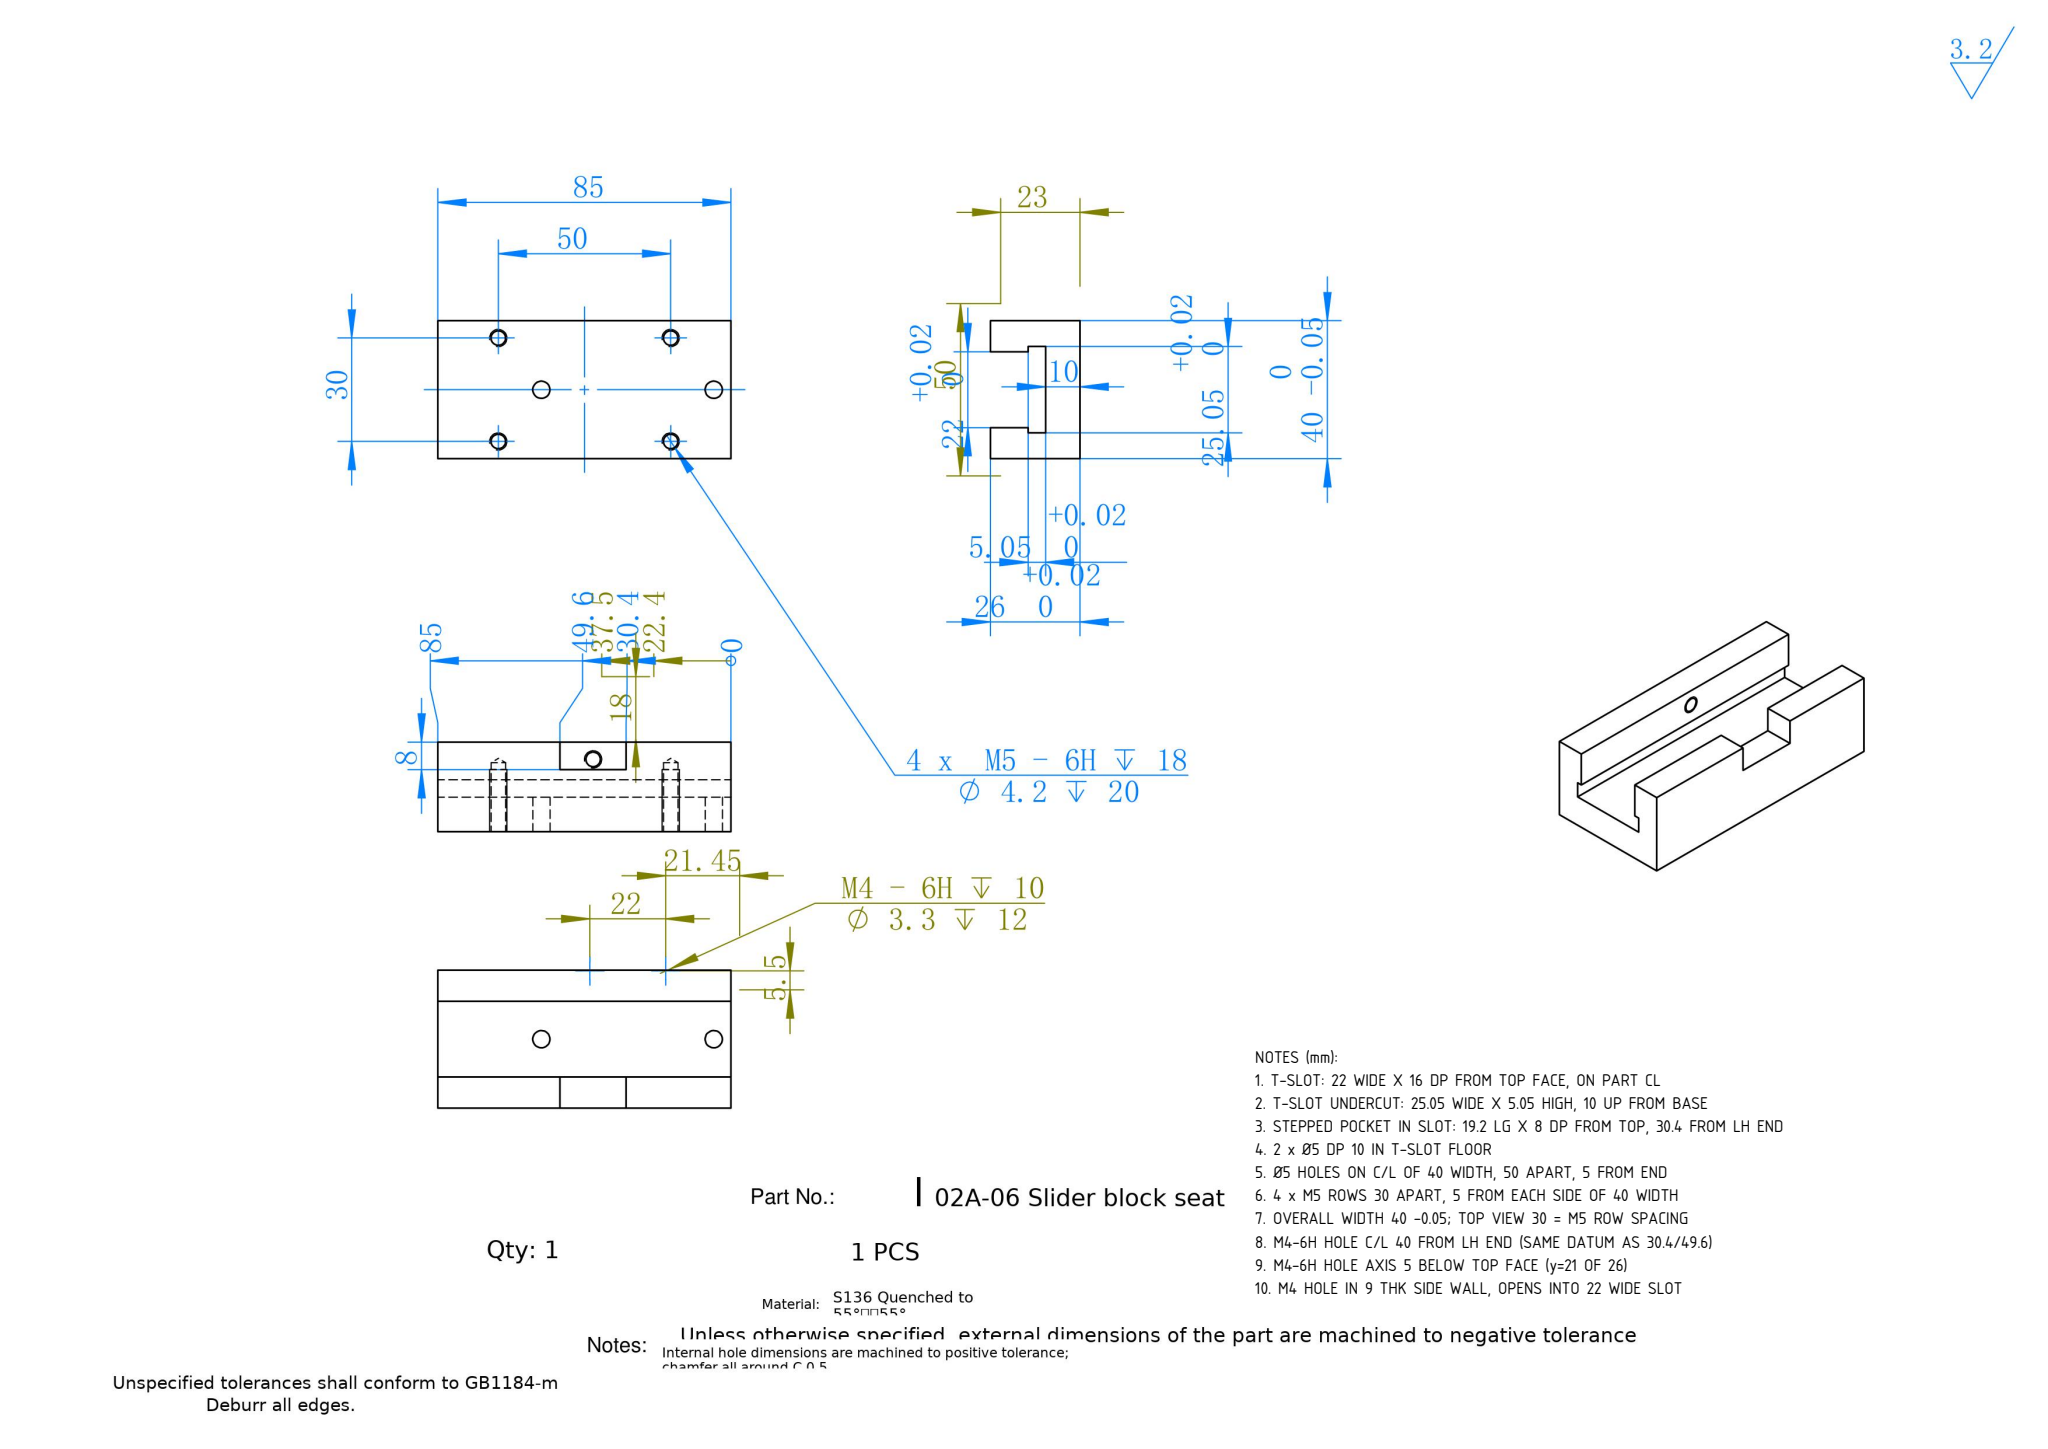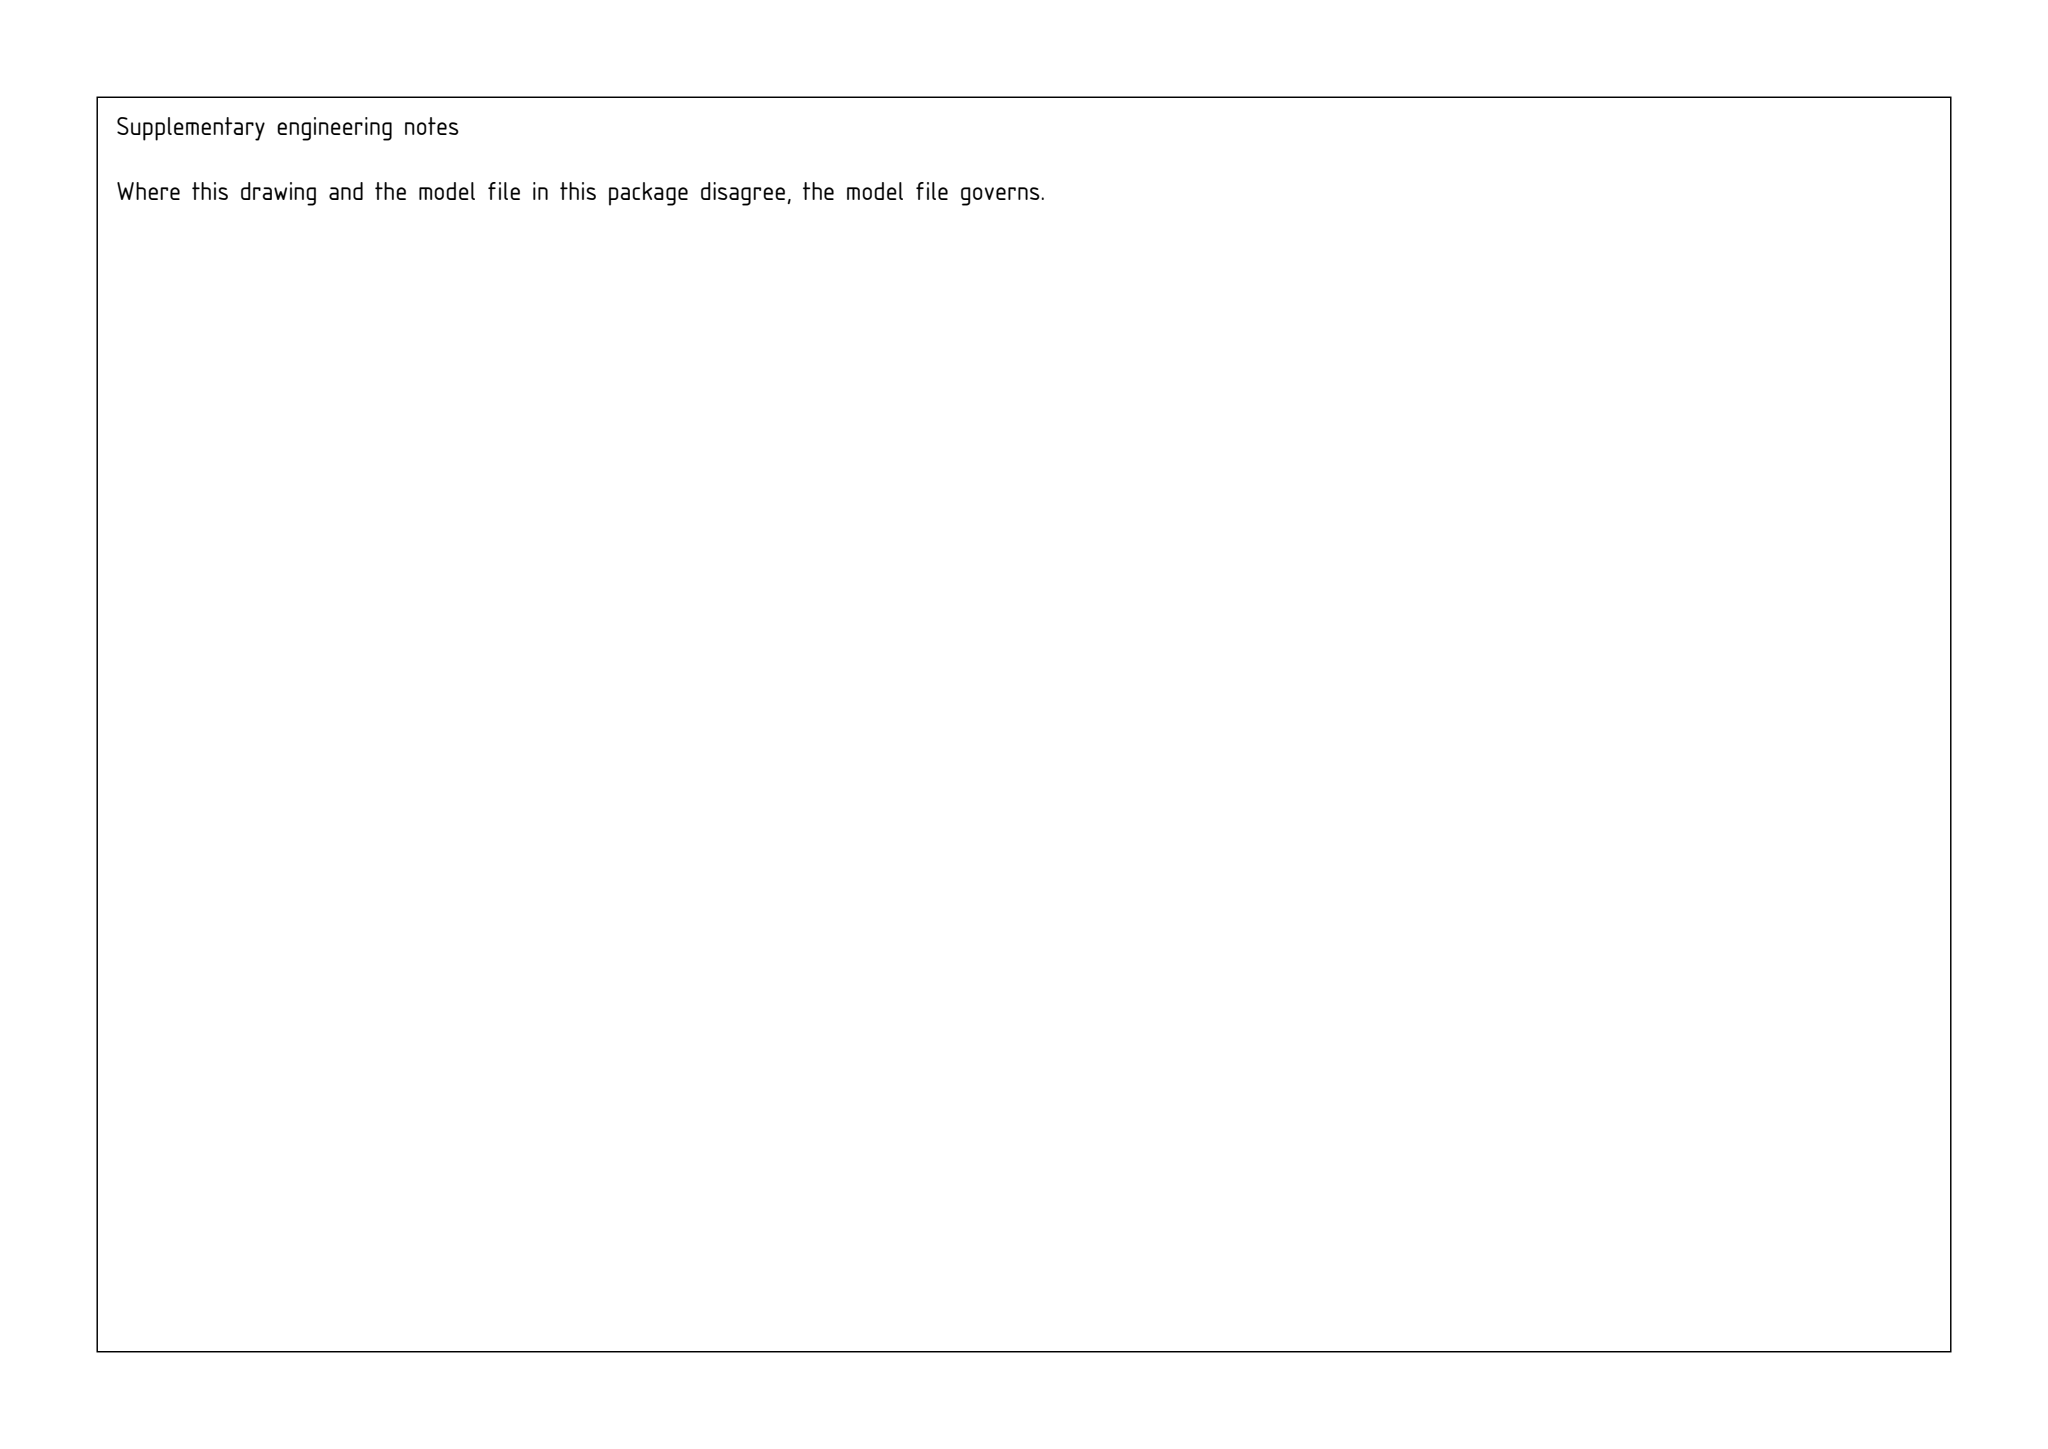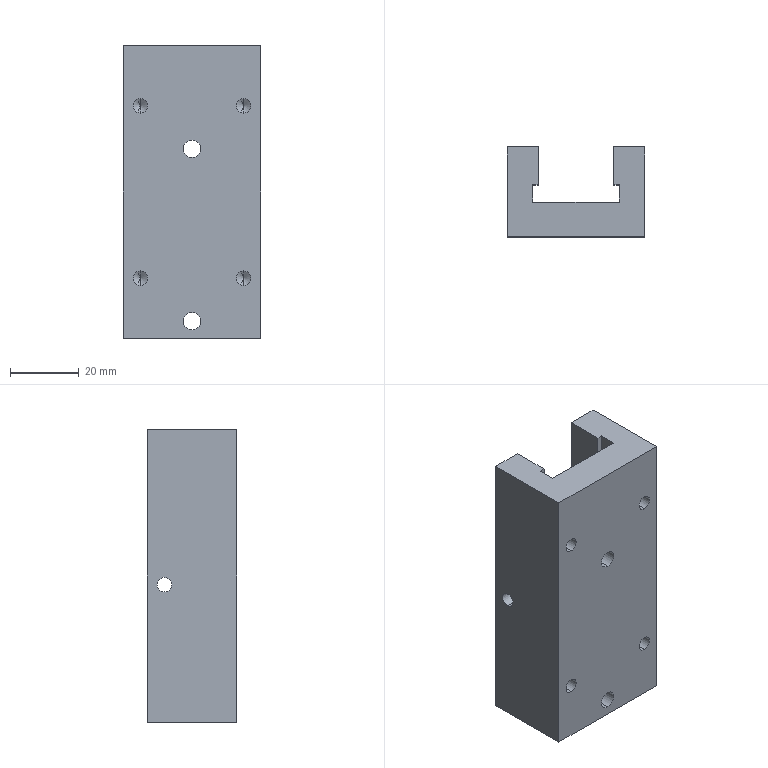Part | SolidWorks | mm | 1 solid | 40 faces | box 40 x 26 x 85 mm | volume 54139 mm3 | plane 18 | cylinder 14 | cone 8 | commonest cylinder face diameters 4.2 x10 5 x4
Drawing notes:
T-SLOT: 22 WIDE X 16 DP FROM TOP FACE, ON PART CL | from the solid: x planes 9.0/31.0 = 22 wide, CL x=20; top face y=26 to slot floor y=10 = 16 dp
T-SLOT UNDERCUT: 25.05 WIDE X 5.05 HIGH, 10 UP FROM BASE | from the solid: x planes 7.48/32.53 = 25.05; y 10.0 to 15.05 = 5.05, base face y=0
STEPPED POCKET IN SLOT: 19.2 LG X 8 DP FROM TOP, 30.4 FROM LH END | from the solid: z planes 30.4/49.6 = 19.2 lg from z=0 end; step floor y=18 vs top y=26 = 8 dp
2 x Ø5 DP 10 IN T-SLOT FLOOR | from the solid: cylinders dia 5.0, axis y, length 10.0, at x=20, z=5 and z=55
Ø5 HOLES ON C/L OF 40 WIDTH, 50 APART, 5 FROM END | from the solid: Ø5 axes at x=20.0 (=40/2), z=5.0 and 55.0 (spacing 50)
4 x M5 ROWS 30 APART, 5 FROM EACH SIDE OF 40 WIDTH | from the solid: Ø4.2 y-axis holes at x=5.0 and x=35.0; bbox x=40.0
OVERALL WIDTH 40 -0.05; TOP VIEW 30 = M5 ROW SPACING | from the solid: bbox_xyz x=40.0; planes x=0.0 and x=40.0; hole rows x=5/35
M4-6H HOLE C/L 40 FROM LH END (SAME DATUM AS 30.4/49.6) | from the solid: Cyl dia4.2 axis X at z=40.0 from z=0 end; z planes 0/30.4/49.6/85 share this datum
M4-6H HOLE AXIS 5 BELOW TOP FACE (y=21 OF 26) | from the solid: Cyl dia4.2 axis X at y=21.0; top face plane y=26.0 -> 26-21=5
M4 HOLE IN 9 THK SIDE WALL, OPENS INTO 22 WIDE SLOT | from the solid: Cyl dia4.2 axis X len 9.0; x planes 0/9.0 and 31.0/40.0 give 9 thk walls, slot 31-9=22
build123d program:
from build123d import *

# Parameters (mm, degrees)
BOSS_EXTRUDE1_DEPTH            = 42.5
CUT_EXTRUDE1_START             = -9
SKETCH3_W                      = 19.2
SKETCH3_H                      = 8
CUT_EXTRUDE1_DEPTH             = 9
M5_TAPPED_HOLE1_D              = 4.2
M5_TAPPED_HOLE1_DEPTH          = 20
M5_TAPPED_HOLE1_TIP            = 1.262
SIZE_MM_DOWEL_PIN_HOLE_0_D     = 5
SIZE_MM_DOWEL_PIN_HOLE_0_DEPTH = 20
SIZE_MM_DOWEL_PIN_HOLE_0_TIP   = 1.502
M5_TAPPED_HOLE2_D              = 4.2


with BuildPart() as part:
    # Sketch1 → Boss-Extrude1 (new, symmetric)
    with BuildSketch(Plane.XY):
        Polygon((-11, 15.05), (-12.525, 15.05), (-12.525, 10), (12.525, 10), (12.525, 15.05), (11, 15.05), (11, 26), (20, 26), (20, 0), (-20, 0), (-20, 26), (-11, 26), align=None)
    extrude(amount=BOSS_EXTRUDE1_DEPTH, both=True)

    # Sketch3 → Cut-Extrude1 (cut)
    with BuildSketch(Plane(origin=(20, 0, 0), x_dir=(0, 0, -1), z_dir=(1, 0, 0)).offset(CUT_EXTRUDE1_START)):
        with Locations((2.5, 22)):
            Rectangle(SKETCH3_W, SKETCH3_H)
    extrude(amount=CUT_EXTRUDE1_DEPTH, mode=Mode.SUBTRACT)

    # M5 Tapped Hole1
    with Locations(Plane.XZ):
        with Locations((-15, -25), (15, -25), (15, 25), (-15, 25)):
            Hole(M5_TAPPED_HOLE1_D / 2, depth=M5_TAPPED_HOLE1_DEPTH)
            with Locations((0, 0, -(M5_TAPPED_HOLE1_DEPTH + M5_TAPPED_HOLE1_TIP / 2))):  # 118° drill point
                Cone(0, M5_TAPPED_HOLE1_D / 2, M5_TAPPED_HOLE1_TIP, mode=Mode.SUBTRACT)

    # Size mm Dowel Pin Hole 0
    with Locations(Plane(origin=(0, 0, 0), x_dir=(-1, 0, 0), z_dir=(0, -1, 0))):
        with Locations((0, -12.5), (0, 37.5)):
            Hole(SIZE_MM_DOWEL_PIN_HOLE_0_D / 2, depth=SIZE_MM_DOWEL_PIN_HOLE_0_DEPTH)
            with Locations((0, 0, -(SIZE_MM_DOWEL_PIN_HOLE_0_DEPTH + SIZE_MM_DOWEL_PIN_HOLE_0_TIP / 2))):  # 118° drill point
                Cone(0, SIZE_MM_DOWEL_PIN_HOLE_0_D / 2, SIZE_MM_DOWEL_PIN_HOLE_0_TIP, mode=Mode.SUBTRACT)

    # M5 Tapped Hole2 (through all)
    with Locations(Plane(origin=(20, 0, 0), x_dir=(0, 0, -1), z_dir=(1, 0, 0))):
        with Locations((2.5, 21)):
            Hole(M5_TAPPED_HOLE2_D / 2)


solid = part.part